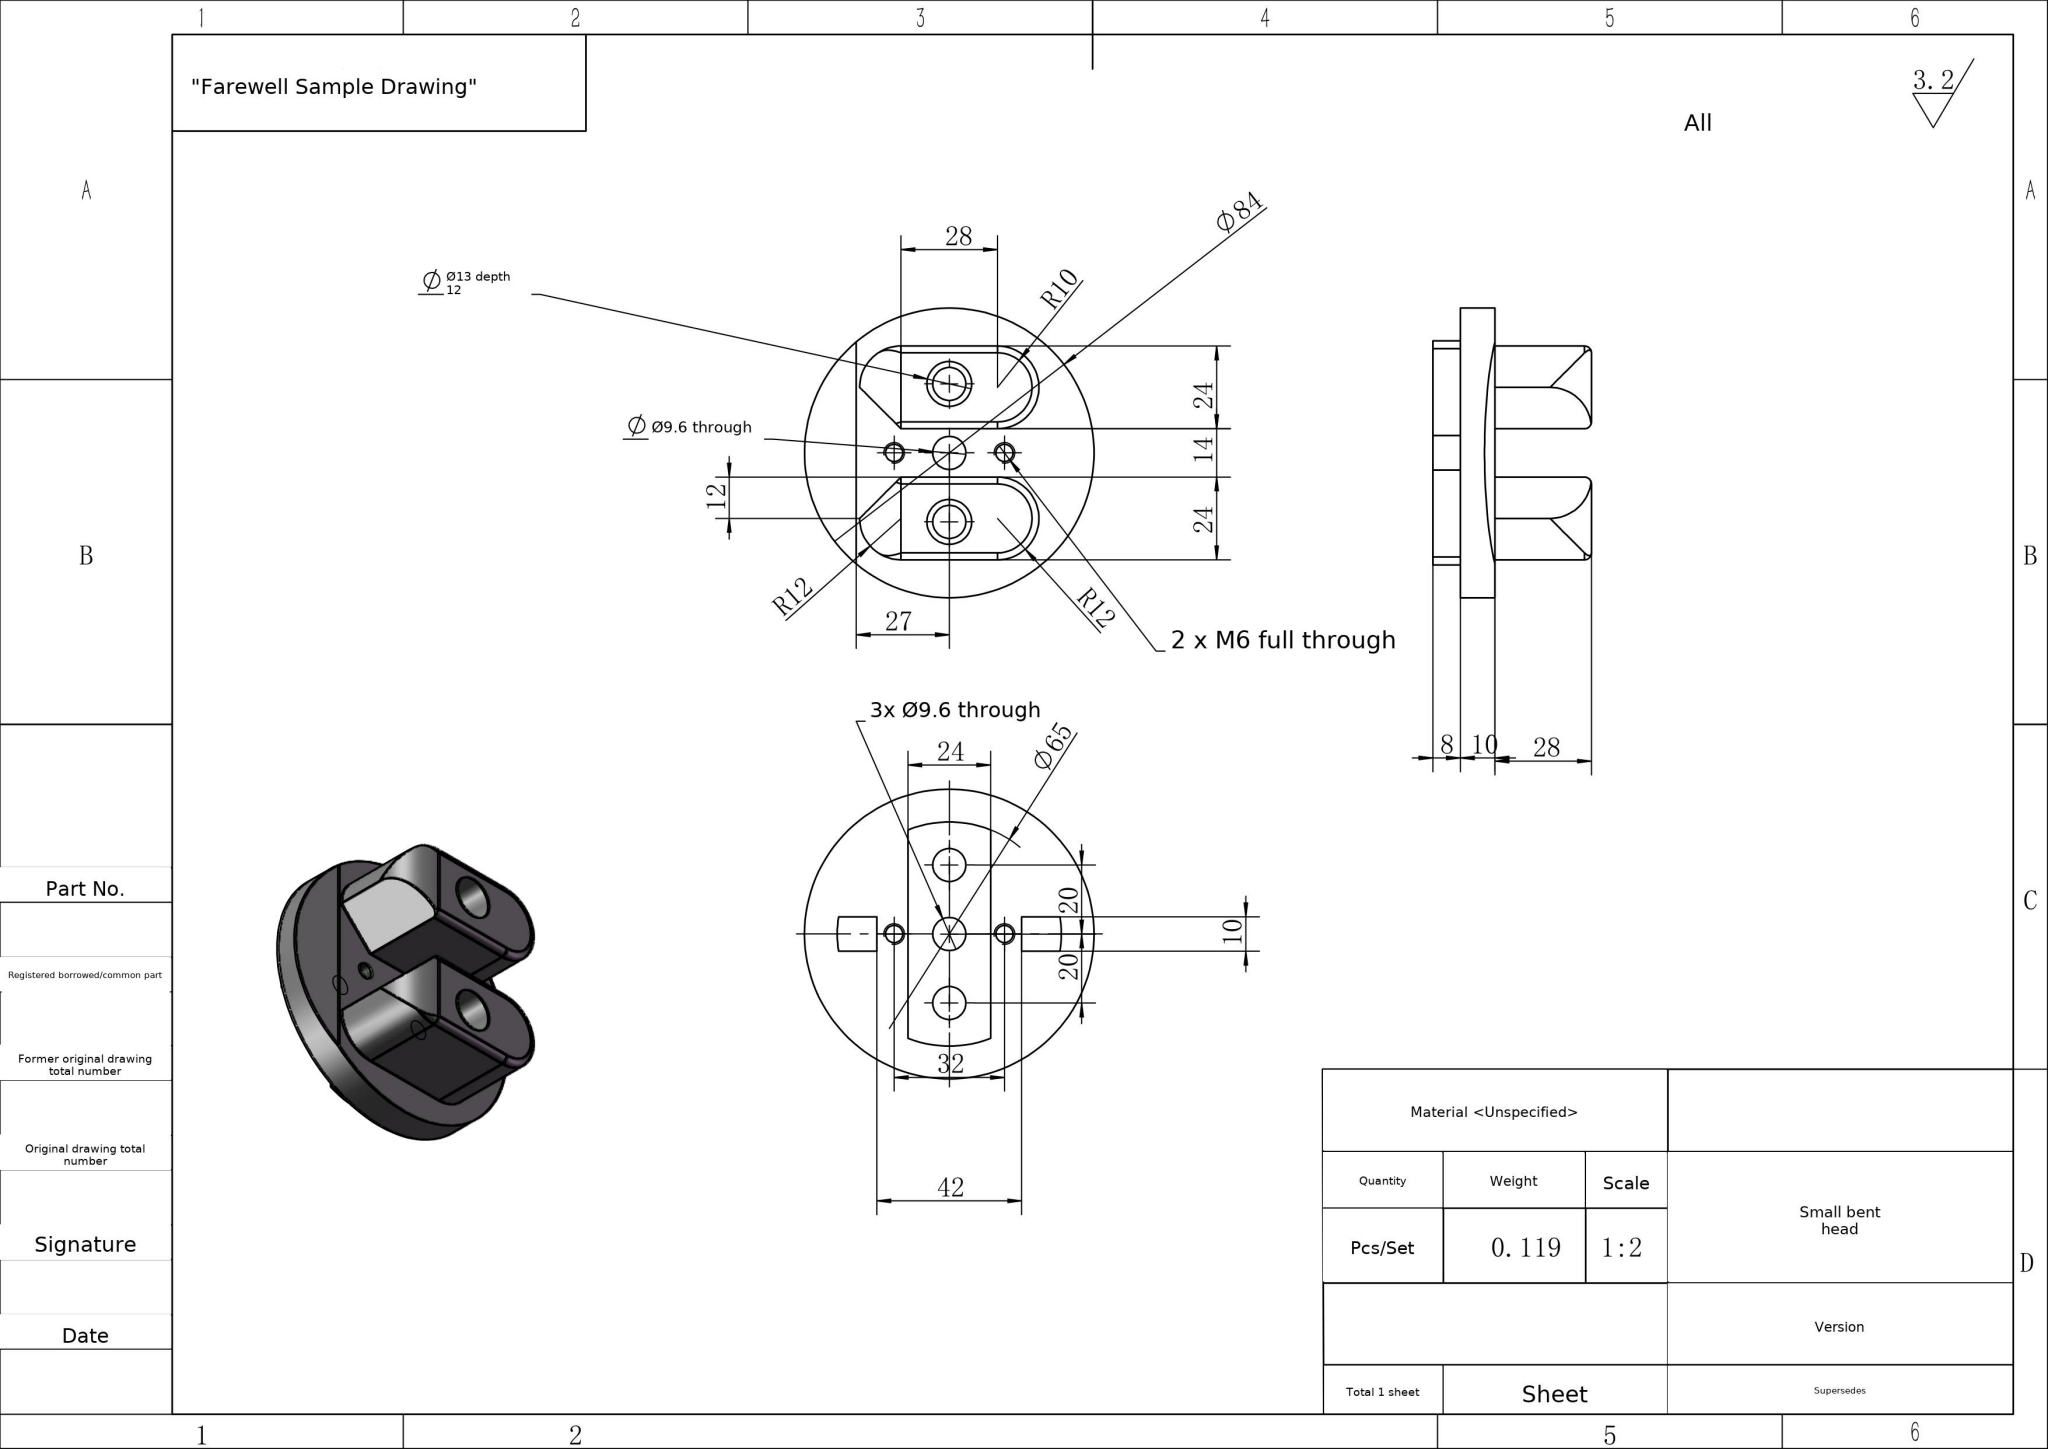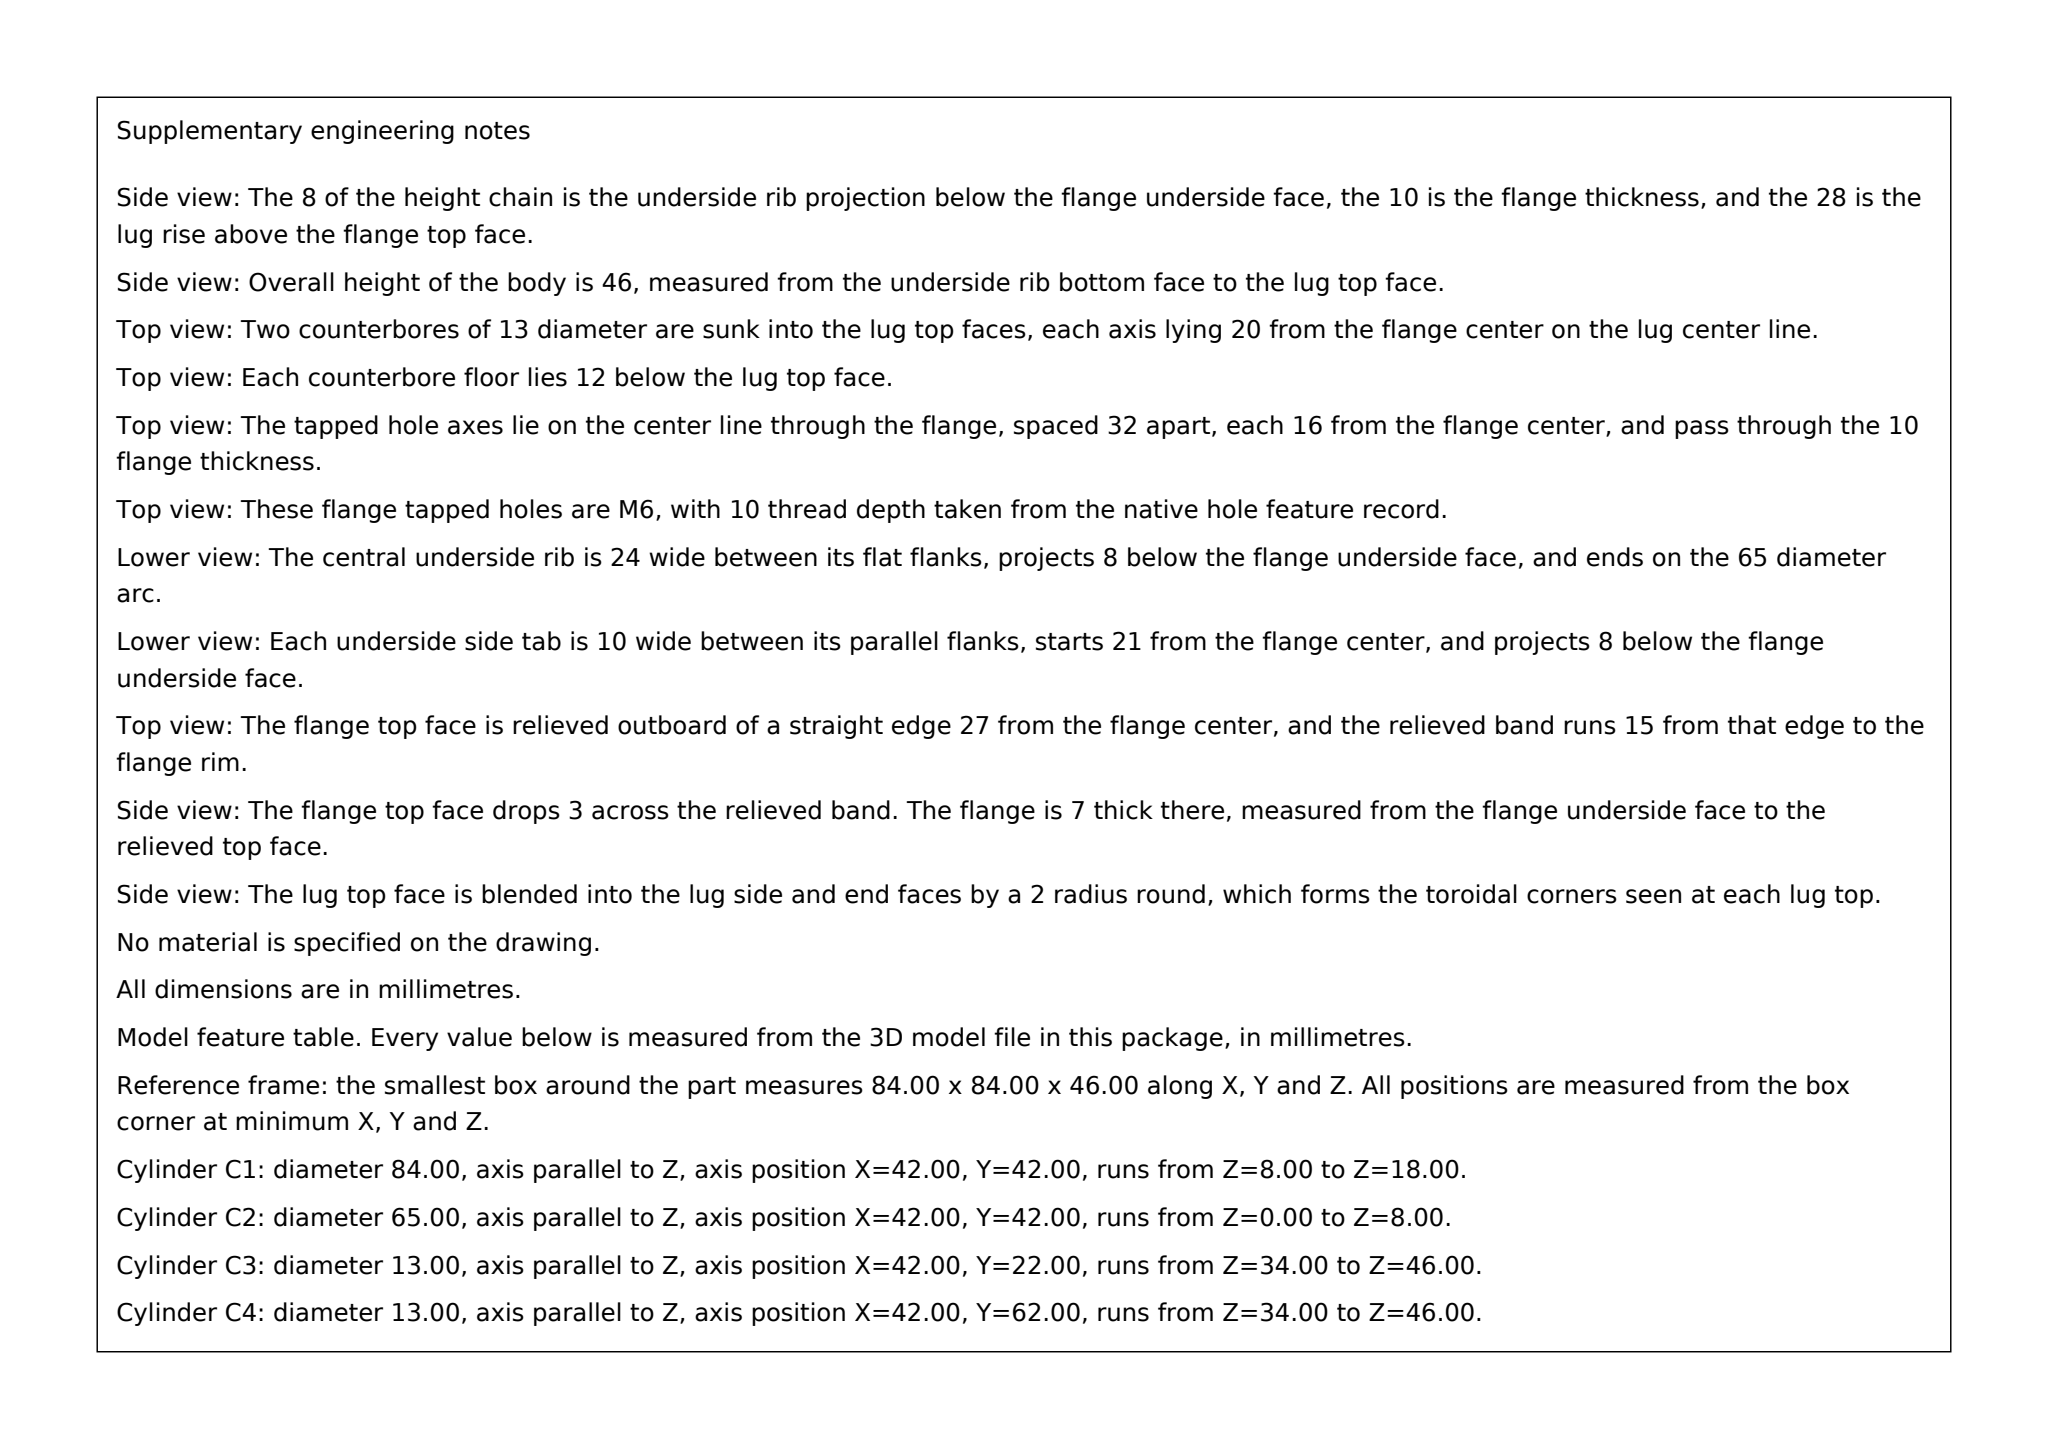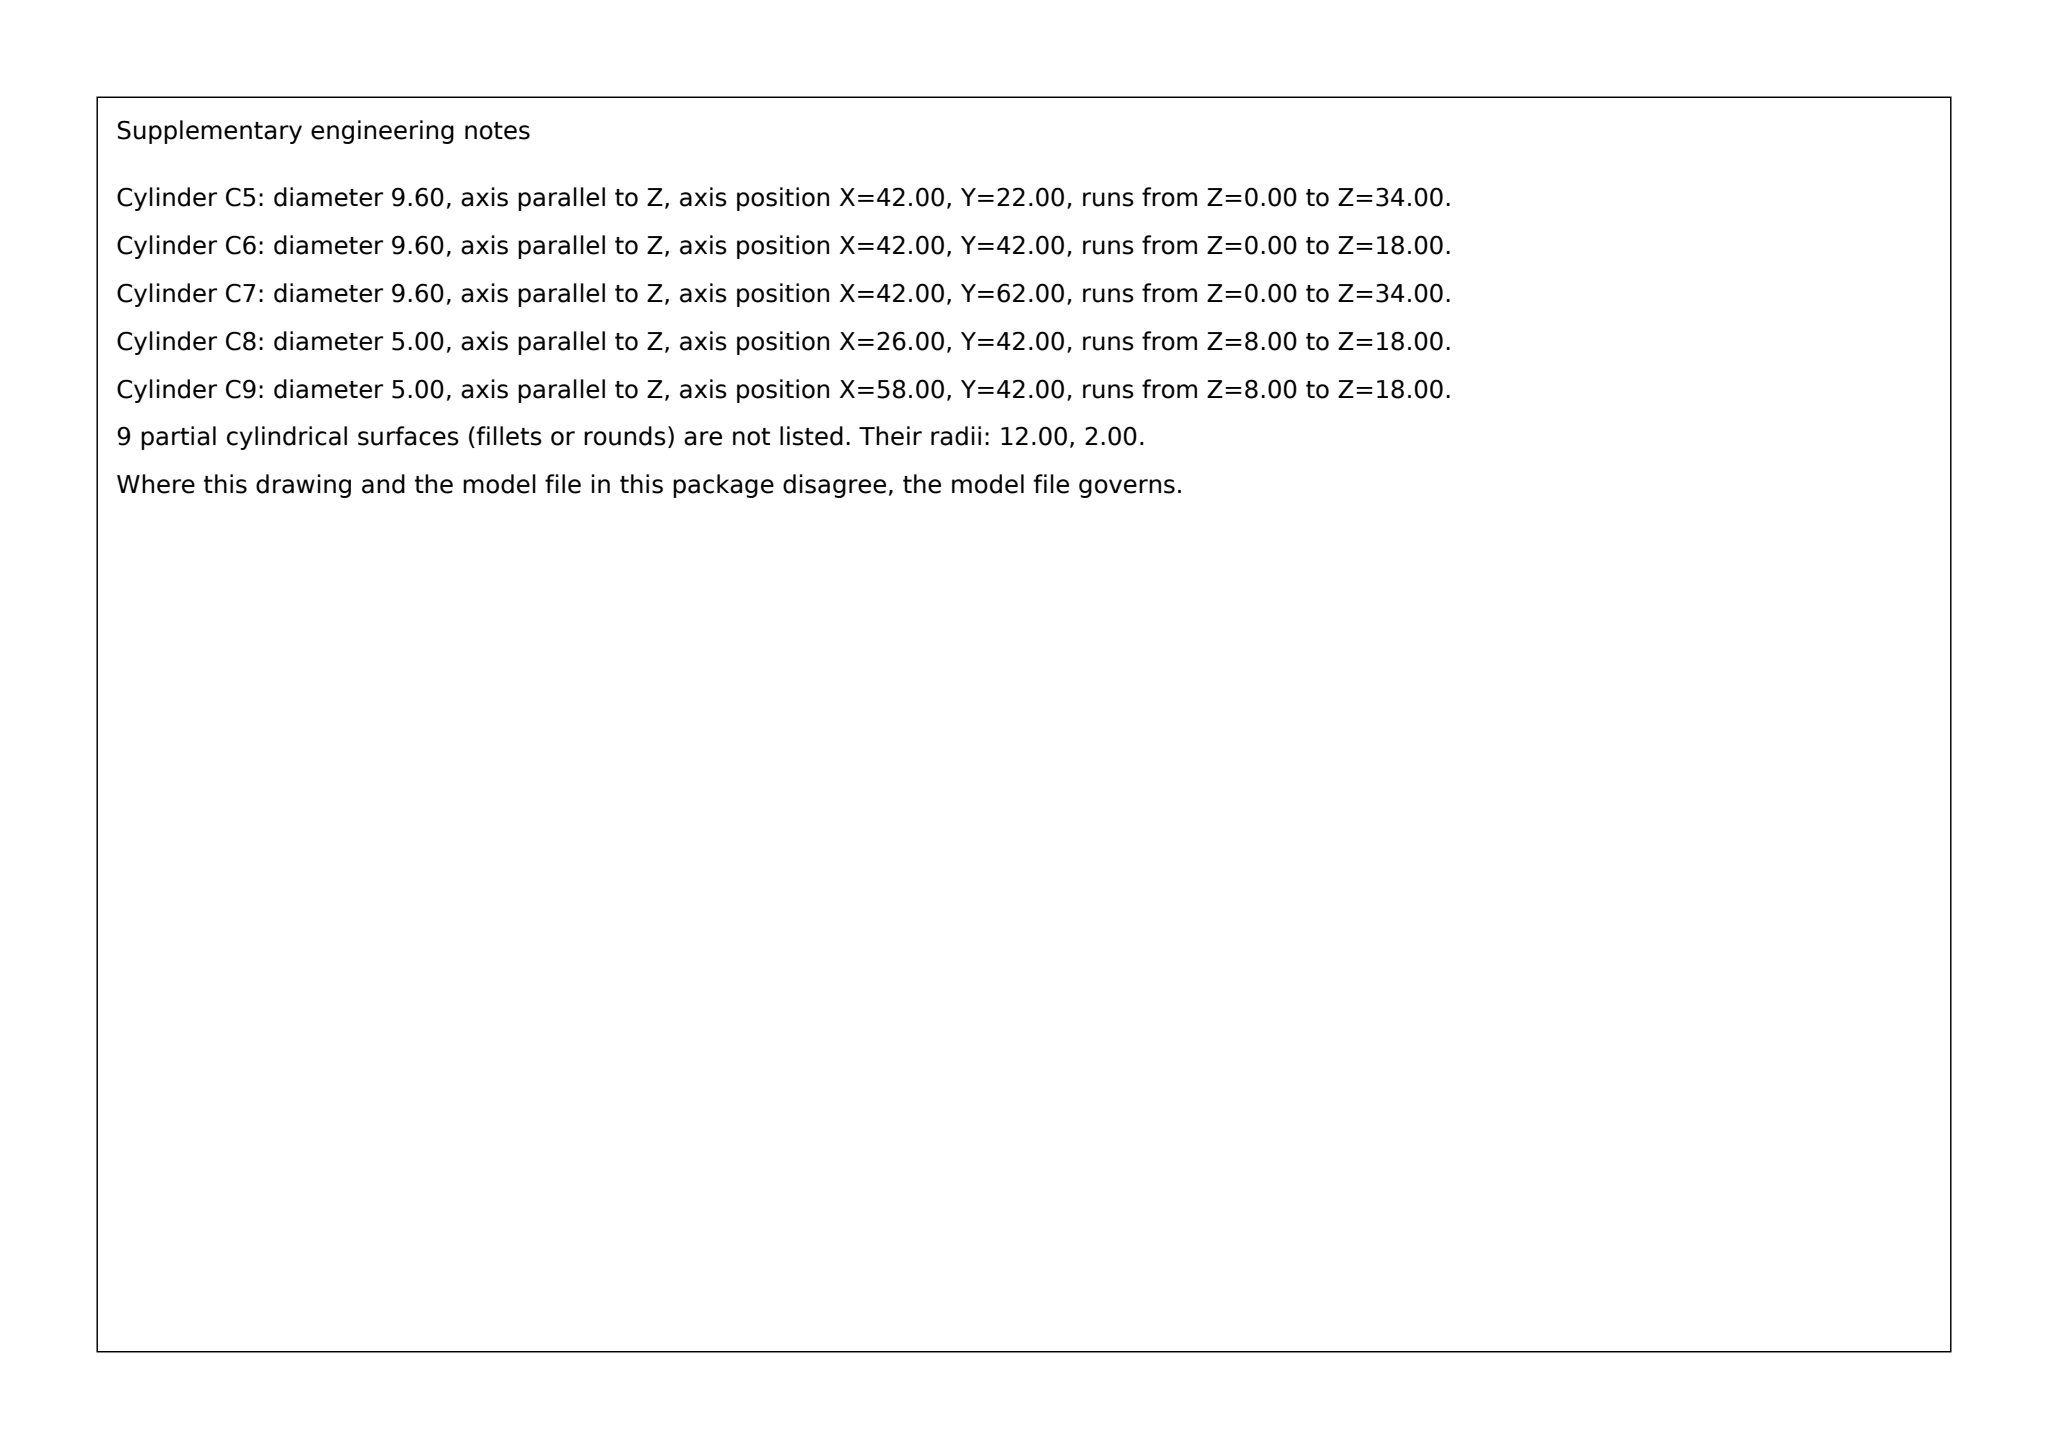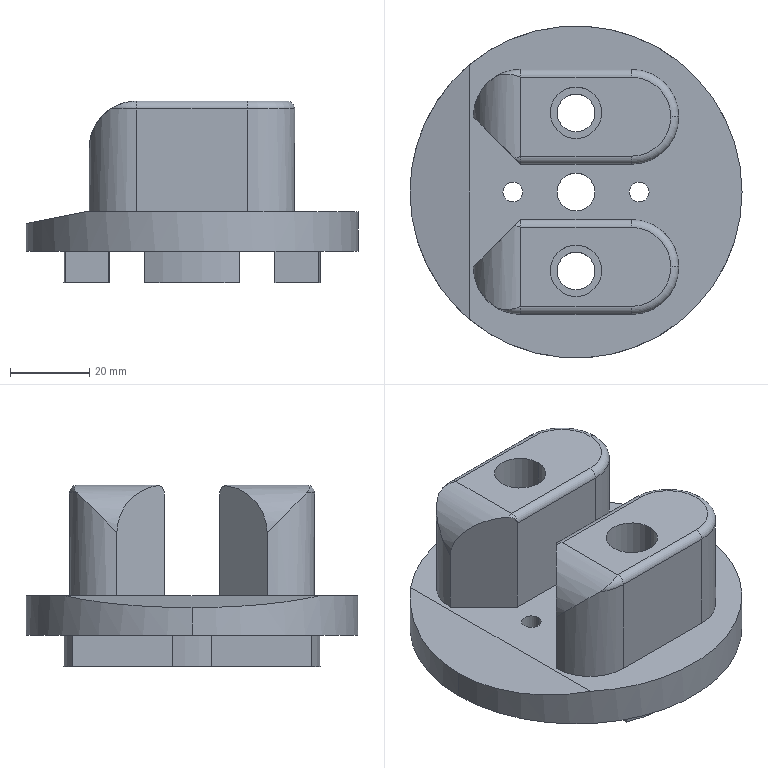Part | SolidWorks | mm | 1 solid | 63 faces | box 84 x 84 x 46 mm | volume 118730 mm3 | cylinder 31 | plane 24 | torus 8 | commonest cylinder face diameters 9.6 x6 24 x6 65 x5 5 x4 13 x4 4 x4 84 x2
Drawing notes:
UNSPECIFIED FILLETS & ROUNDS R2 (8 PL), INCL FORK ARM TIP EDGES | from the solid: fillet_radii: [[2.0, 8]] - eight 2 mm edge rounds, no other radii besides called-out R10/R12
R12 SCOOP: CL 12 FROM ARM END, 14 OFF PART CL, FULL ARM WIDTH | from the solid: cylinders: [24.0 dia, axis x, pos (y=null skipped) -> entry [24.0,"y",[28.0,null,34.0],21.3] = R12 concave cut, axis along Y at x=28, z=34, cut length 21.3 across 24-wide arm; arm end face z=46 (46-34=12), part CL x=42 (42-28=14), flange face z=18 (34-18=16); fillet_radii 2.0 at cut corners
2X RECTANGULAR POCKET 9 WIDE (ACROSS) X 10 WIDE, 8 DEEP: POCKETS OPEN AT THE REAR (Ø65) FACE AND RUN 8 INWARD; FLOOR COPLANAR WITH THE Ø84 FLANGE REAR FACE, LEAVING A 10 THICK WEB TO THE FORK-SIDE FACE (TOTAL PLATE 18 FROM REAR FACE TO FORK-SIDE FACE) | from the solid: pocket walls at x=21/30 and x=54/63 with y=37/47; z planes 0 (rear face) and 8 (pocket floor / flange rear face); z plane 18 = fork-side face; Ø5 (M6) holes length 10 = remaining web
Ø13 COUNTERBORE DEPTH 12 - 2 PLACES, ONE AT EACH Ø9.6 HOLE LOCATED 20 EITHER SIDE OF THE PART CENTRELINE, COUNTERBORED FROM THE FORK ARM END FACE | from the solid: cylinders dia 13.0, axis z, at (42,22) and (42,62), length 12, matching the two 9.6 dia holes at y=22 and y=62 (part centre y=42); arm end plane z=46 with cbore floors at z=34
build123d program:
from build123d import *

# Parameters (mm, degrees)
SKETCH1_R           = 42
BOSS_EXTRUDE1_DEPTH = 10
SKETCH2_R           = 4.8
CUT_EXTRUDE1_DEPTH  = 14.5
SKETCH4_R           = 4.8
BOSS_EXTRUDE3_DEPTH = 8
BOSS_EXTRUDE4_DEPTH = 28
SKETCH7_R           = 4.8
CUT_EXTRUDE4_DEPTH  = 66.666
SKETCH8_R           = 6.5
CUT_EXTRUDE5_DEPTH  = 12
FILLET2_R           = 2
SKETCH9_R           = 4.8
CUT_EXTRUDE6_DEPTH  = 66.666
CUT_EXTRUDE7_DEPTH  = 93.396
CUT_EXTRUDE8_REACH  = 77.127
M6_TAPPED_HOLE1_D   = 5
CUT_EXTRUDE9_DEPTH  = 50


with BuildPart() as part:
    # Sketch1 → Boss-Extrude1 (new body)
    with BuildSketch(Plane.XY):
        Circle(SKETCH1_R)
    extrude(amount=BOSS_EXTRUDE1_DEPTH)

    # Sketch2 → Cut-Extrude1 (cut)
    with BuildSketch(Plane.XY.offset(10)):
        with Locations((0, 20)):
            Circle(SKETCH2_R)
        with Locations((0, -20)):
            Circle(SKETCH2_R)
    extrude(amount=-CUT_EXTRUDE1_DEPTH, mode=Mode.SUBTRACT)

    # Sketch4 → Boss-Extrude3 (add)
    # profile 1 of 3: a face of its own
    with BuildSketch(Plane(origin=(0, 0, 0), x_dir=(-1, 0, 0), z_dir=(0, 0, -1))):
        with BuildLine():
            Line((-12, 30.203), (-12, -30.203))
            ThreePointArc((-12, -30.203), (0, -32.5), (12, -30.203))
            Line((12, -30.203), (12, 30.203))
            ThreePointArc((12, 30.203), (0, 32.5), (-12, 30.203))
        make_face()
        with Locations(Location((0, -20, 0), (0, 0, 180))):
            Circle(SKETCH4_R, mode=Mode.SUBTRACT)
        with Locations(Location((0, 20, 0), (0, 0, 180))):
            Circle(SKETCH4_R, mode=Mode.SUBTRACT)
    # profile 2 of 3: a face of its own
    with BuildSketch(Plane(origin=(0, 0, 0), x_dir=(-1, 0, 0), z_dir=(0, 0, -1))):
        with BuildLine():
            Line((21, 5), (32.113, 5))
            ThreePointArc((32.113, 5), (32.5, 0), (32.113, -5))
            Line((32.113, -5), (21, -5))
            Line((21, -5), (21, 5))
        make_face()
    # profile 3 of 3: a face of its own
    with BuildSketch(Plane(origin=(0, 0, 0), x_dir=(-1, 0, 0), z_dir=(0, 0, -1))):
        with BuildLine():
            Line((-32.113, 5), (-21, 5))
            Line((-21, 5), (-21, -5))
            Line((-21, -5), (-32.113, -5))
            ThreePointArc((-32.113, -5), (-32.5, 0), (-32.113, 5))
        make_face()
    extrude(amount=BOSS_EXTRUDE3_DEPTH)

    # Sketch6 → Boss-Extrude4 (add)
    with BuildSketch(Plane.XY.offset(10)):
        with BuildLine():
            Line((-14, 31), (14, 31))
            ThreePointArc((14, 31), (26, 19), (14, 7))
            Line((14, 7), (-14, 7))
            ThreePointArc((-14, 7), (-26, 19), (-14, 31))
        make_face()
        with BuildLine():
            Line((-14, -7), (14, -7))
            ThreePointArc((14, -7), (26, -19), (14, -31))
            Line((14, -31), (-14, -31))
            ThreePointArc((-14, -31), (-26, -19), (-14, -7))
        make_face()
    extrude(amount=BOSS_EXTRUDE4_DEPTH)

    # Sketch7 → Cut-Extrude4 (cut, through all)
    with BuildSketch(Plane(origin=(0, 0, 10), x_dir=(-1, 0, 0), z_dir=(0, 0, -1))):
        with Locations(Location((0, 20, 0), (0, 0, 180))):
            Circle(SKETCH7_R)
        with Locations(Location((0, -20, 0), (0, 0, 180))):
            Circle(SKETCH7_R)
    extrude(amount=-CUT_EXTRUDE4_DEPTH, mode=Mode.SUBTRACT)

    # Sketch8 → Cut-Extrude5 (cut)
    with BuildSketch(Plane.XY.offset(38)):
        with Locations((0, 20)):
            Circle(SKETCH8_R)
        with Locations((0, -20)):
            Circle(SKETCH8_R)
    extrude(amount=-CUT_EXTRUDE5_DEPTH, mode=Mode.SUBTRACT)

    # Fillet2
    fillet2_edges = [part.edges().sort_by_distance(p)[0] for p in [
        (-26, 19, 38),
        (0, 7, 38),
        (26, 19, 38),
        (0, 31, 38),
        (-26, -19, 38),
        (0, -31, 38),
        (26, -19, 38),
        (0, -7, 38),
    ]]
    fillet(fillet2_edges, radius=FILLET2_R)

    # Sketch9 → Cut-Extrude6 (cut, through all)
    with BuildSketch(Plane.XY.offset(10)):
        Circle(SKETCH9_R)
    extrude(amount=-CUT_EXTRUDE6_DEPTH, mode=Mode.SUBTRACT)

    # Sketch10 → Cut-Extrude7 (cut, through all)
    with BuildSketch(Plane.XZ.offset(31)):
        with BuildLine():
            Line((-26, 26), (-26, 38))
            Line((-26, 38), (-14, 38))
            ThreePointArc((-14, 38), (-22.485, 34.485), (-26, 26))
        make_face()
    extrude(amount=-CUT_EXTRUDE7_DEPTH, mode=Mode.SUBTRACT)

    # Cut-Extrude8: up to this face of the body (flat: up to its plane)
    cut_extrude8_end = Plane(part.part.faces().sort_by_distance((-40.812, 0, 10))[0])
    # Sketch11 → Cut-Extrude8 (cut, up to the picked face)
    with BuildSketch(Plane.XY.offset(38), mode=Mode.PRIVATE) as cut_extrude8_sk1:
        Polygon((-26, 19), (-7, 0), (-26, -19), align=None)
    cut_extrude8_tool1 = split(extrude(cut_extrude8_sk1.sketch, amount=-CUT_EXTRUDE8_REACH, mode=Mode.PRIVATE), bisect_by=cut_extrude8_end, keep=Keep.BOTH, mode=Mode.PRIVATE)
    add(cut_extrude8_tool1.solids().sort_by(Axis((-19.667, 0, 38), (0, 0, -1)))[0], mode=Mode.SUBTRACT)

    # M6 Tapped Hole1 (through all)
    with Locations(Plane(origin=(0, 0, 0), x_dir=(-1, 0, 0), z_dir=(0, 0, -1))):
        with Locations((-16, 0), (16, 0)):
            Hole(M6_TAPPED_HOLE1_D / 2)

    # Sketch14 → Cut-Extrude9 (cut, symmetric)
    with BuildSketch(Plane(origin=(0, 0, 0), x_dir=(1, 0, 0), z_dir=(0, 1, 0))):
        Polygon((-42, -7), (-27, -10), (-42, -10), align=None)
    extrude(amount=CUT_EXTRUDE9_DEPTH, both=True, mode=Mode.SUBTRACT)


solid = part.part